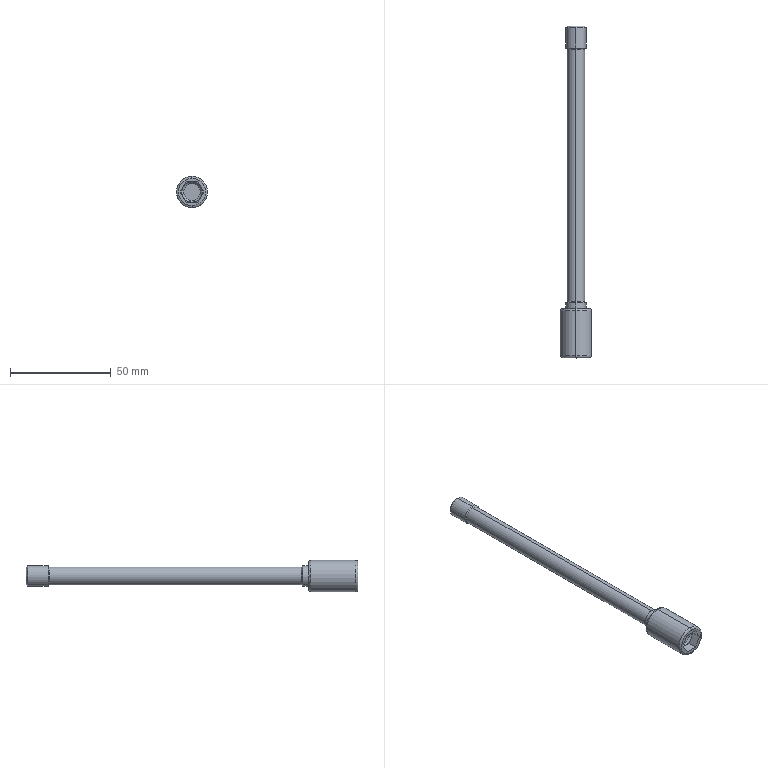Component | SolidWorks | SC-80x75(000)-1_4-1 | 1 solid | 38 faces | volume 12478 mm3 | plane 16 | cylinder 10 | cone 8 | spline 4 | commonest cylinder face diameters 10 x4 8.9 x2 15.5 x2 8.376 x2